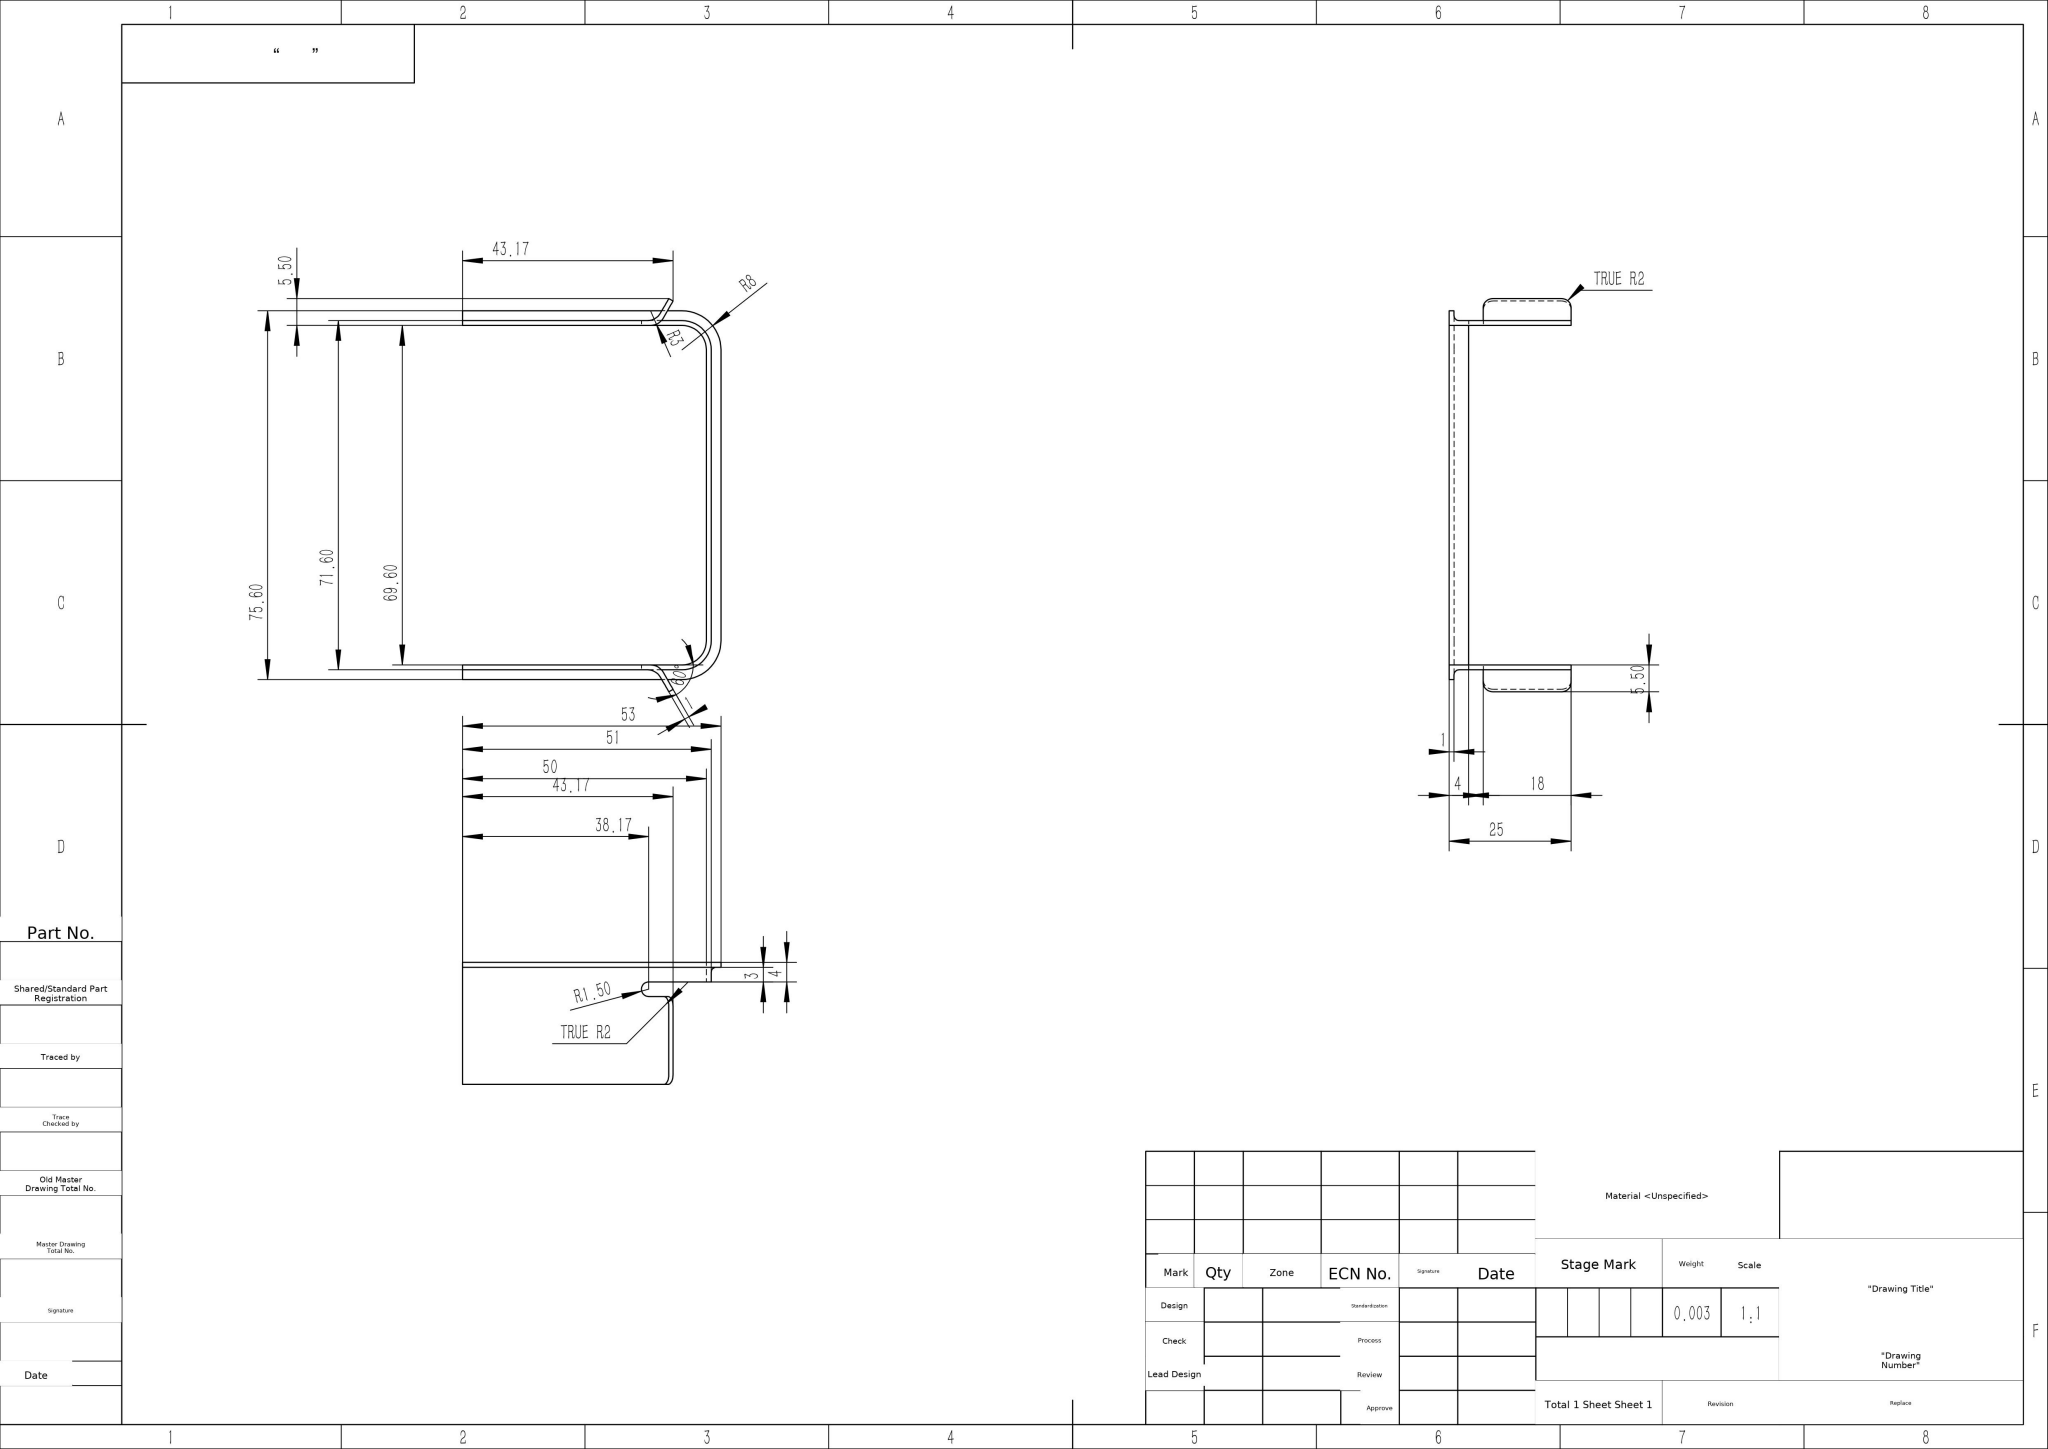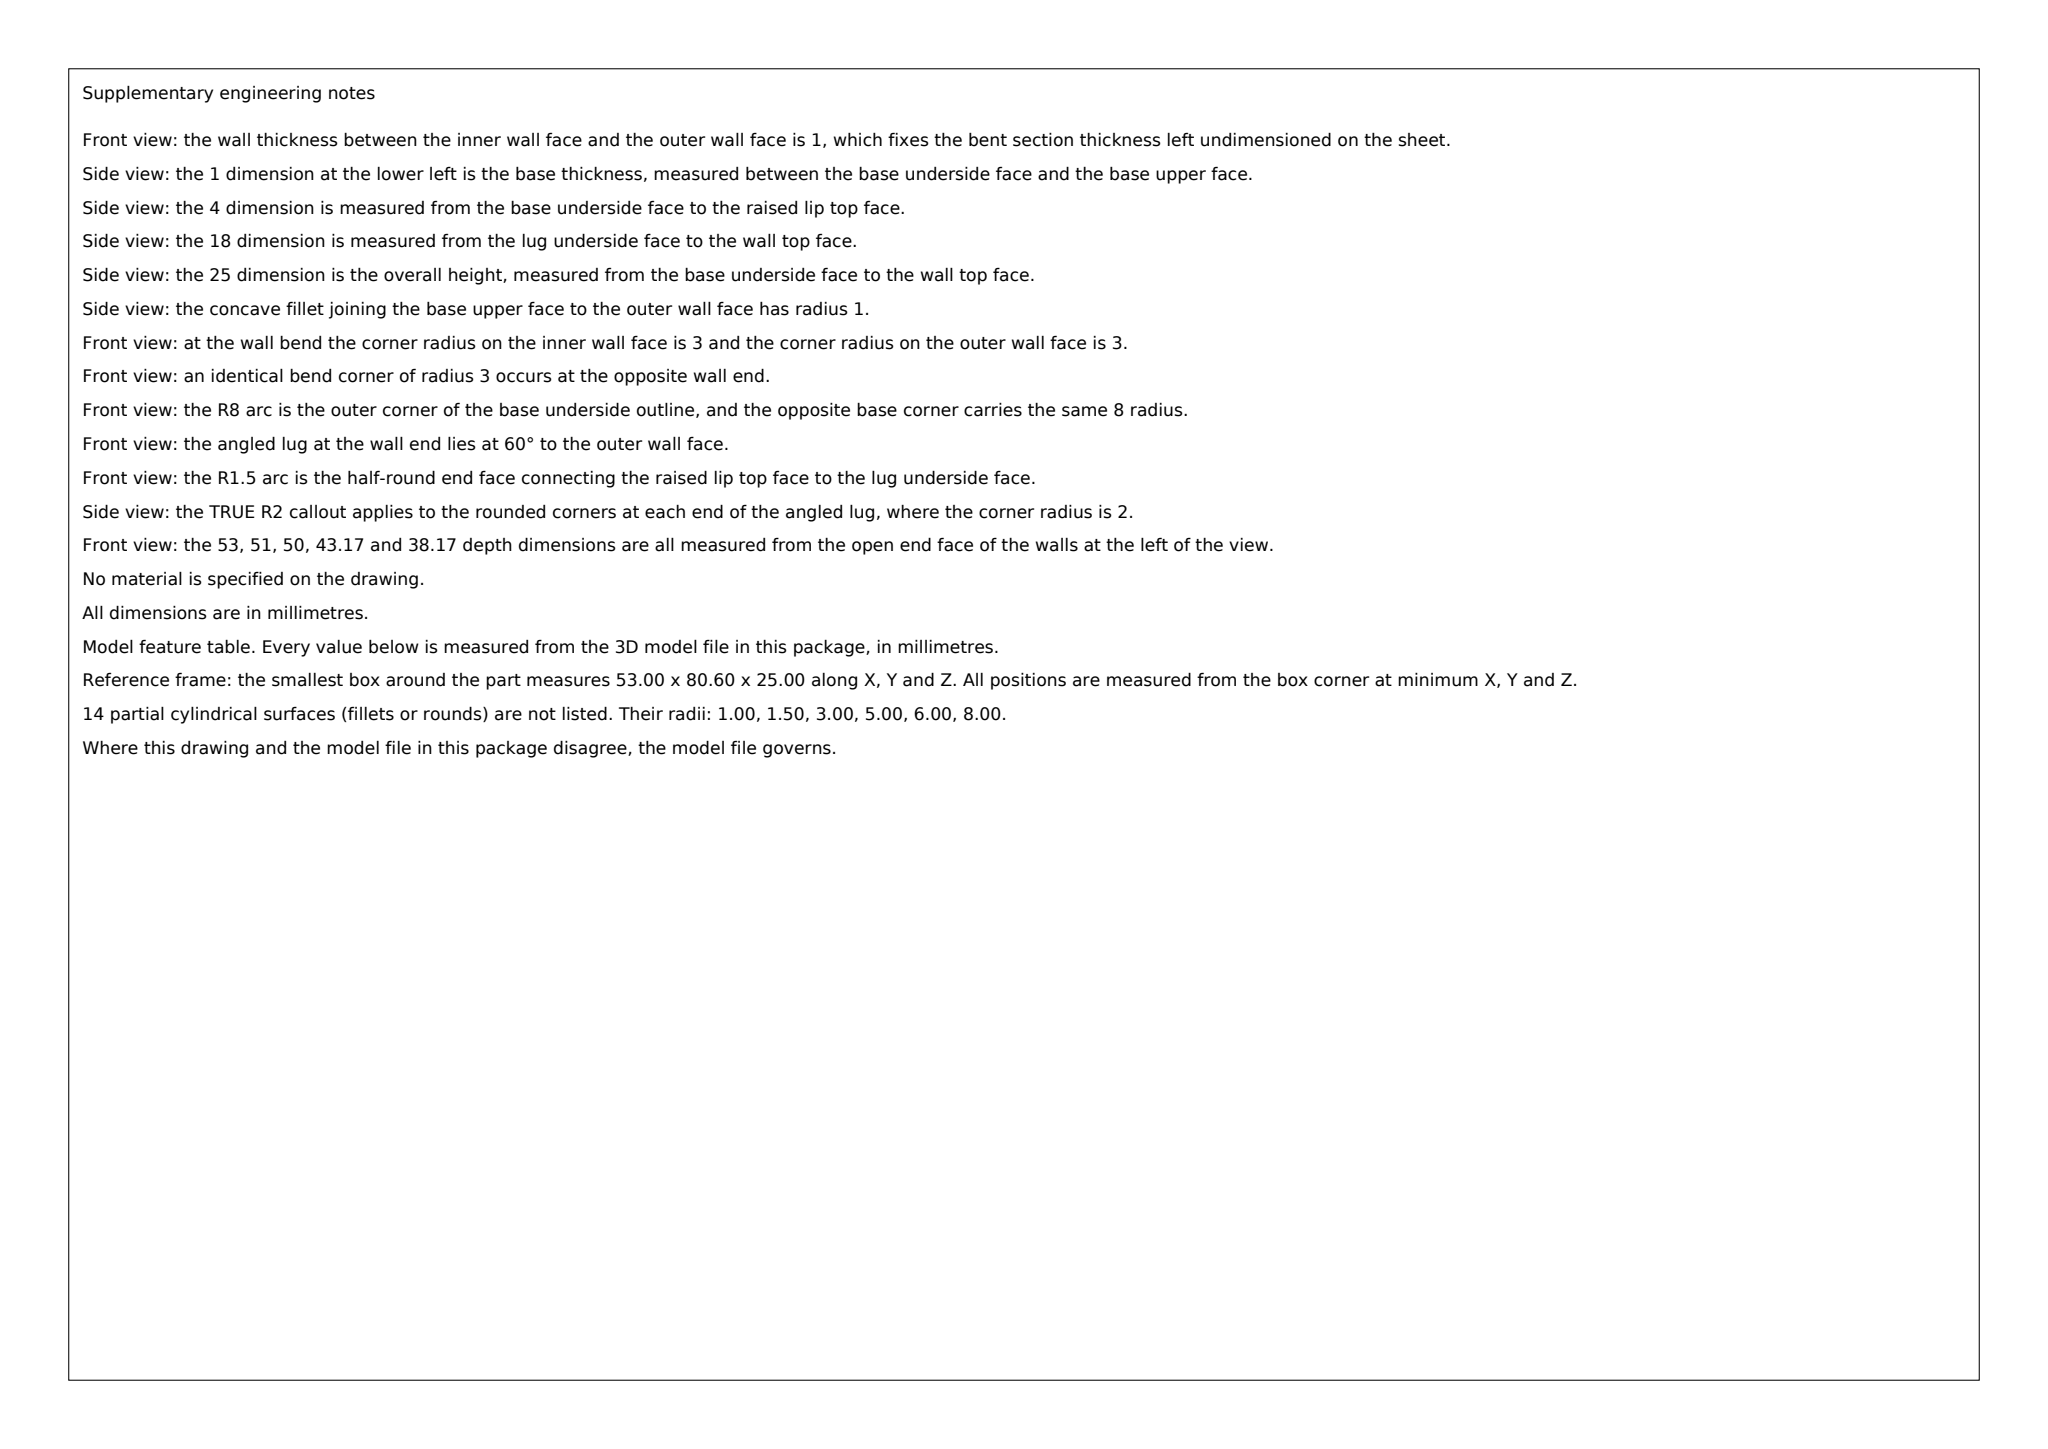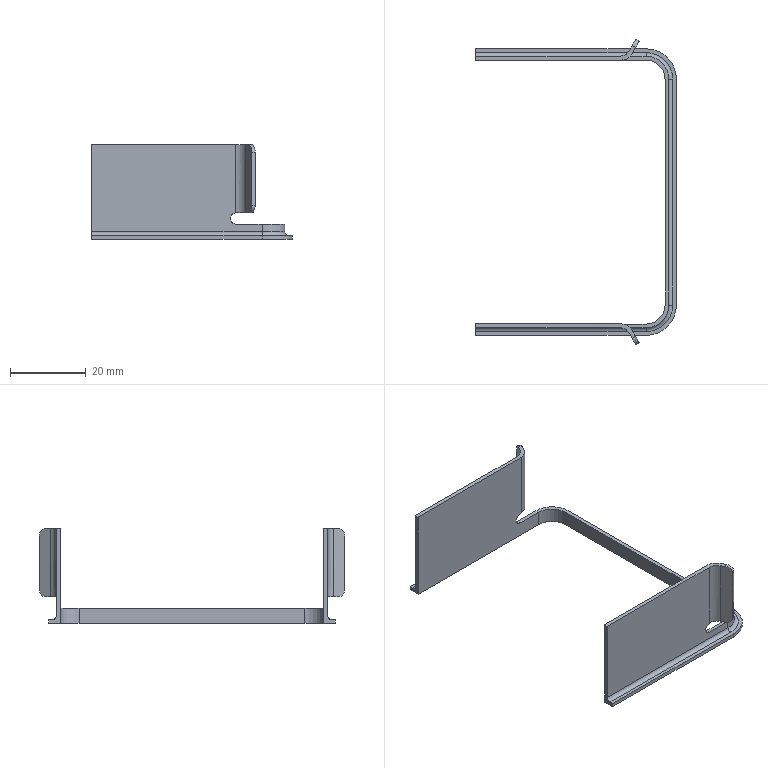Part | SolidWorks | mm | 1 solid | 49 faces | box 53 x 80.6 x 25 mm | volume 2903 mm3 | plane 26 | cylinder 21 | torus 2 | commonest cylinder face diameters 6 x6 4 x4 2 x3 10 x2 16 x2 12 x2 3 x2
Drawing notes:
2X STEPPED HOLE: Ø10 DP 4, C'BORE Ø12 DP 2, C'BORE Ø16 DP 1 | from the solid: cyl Ø10 z ↧4 at (45,10.5)&(45,70.1); Ø12 ↧2 same axes; Ø16 ↧1 same axes
STEPPED HOLES 45 FROM END FACE; 10.5 & 70.1 FROM FLANGE EDGE | from the solid: Ø10 axes at x=45, y=10.5 and y=70.1 from bbox min corner (x=0 end face, y=0 edge)
STEPPED HOLE C/C SPACING 59.6 | from the solid: 70.1 - 10.5 = 59.6 between Ø10 axes
OVERALL WIDTH 80.6 ACROSS BOTH 5.50 FLANGES | from the solid: bbox_xyz y = 80.6; y-planes at 2.5/4.5/5.5 and 75.1/76.1/78.1